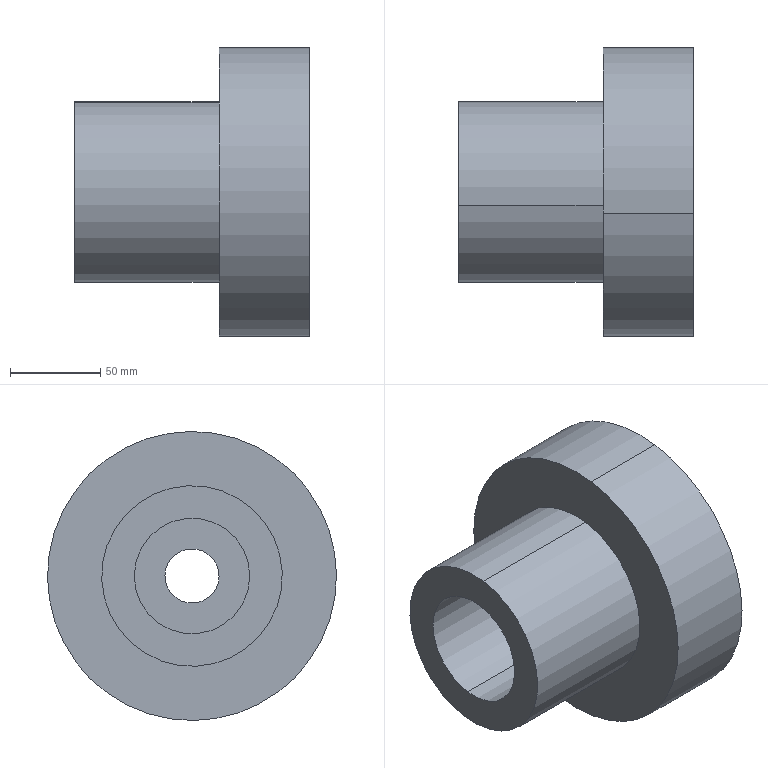Component | SolidWorks | Piston-1 | 1 solid | 18 faces | box 130 x 160 x 160 mm | volume 1255299 mm3 | cylinder 12 | plane 6 | commonest cylinder face diameters 100 x4 30 x2 34 x2 160 x2 64 x2
build123d program:
from build123d import *

# Parameters (mm, degrees)
M30_TAPPED_HOLE1_D     = 30
M30_TAPPED_HOLE1_DEPTH = 115


with BuildPart() as part:
    # Sketch1 → Revolve1 (revolve)
    with BuildSketch(Plane(origin=(0, 0, 0), x_dir=(1, 0, 0), z_dir=(0, 1, 0))):
        Polygon((10, 61), (32, 61), (32, 130), (50, 130), (50, 50), (80, 50), (80, 0), (50, 0), (50, 15), (17, 15), (17, 45), (10, 45), align=None)
    revolve(axis=Axis((0, 0, 0), (0, 0, -1)))

    # M30 Tapped Hole1
    with Locations(Plane.XY.offset(-15)):
        with Locations((0, 0)):
            Hole(M30_TAPPED_HOLE1_D / 2, depth=M30_TAPPED_HOLE1_DEPTH)


solid = part.part

# Placed as in the assembly
solid = solid.moved(Location((-28.66, 0, 0), (0, 90, 0)))
STEP:
#1=CARTESIAN_POINT('',(-3.53,0.08713,-0.5841));
#2=VERTEX_POINT('',#1);
#3=CARTESIAN_POINT('',(-3.53,-0.08713,0.5841));
#4=VERTEX_POINT('',#3);
#5=CARTESIAN_POINT('',(-3.53,-0.,0.));
#6=DIRECTION('',(-1.,-0.,0.));
#7=DIRECTION('',(0.,-0.1475,0.9891));
#8=AXIS2_PLACEMENT_3D('',#5,#6,#7);
#9=CIRCLE('',#8,0.5906);
#10=EDGE_CURVE('',#2,#4,#9,.T.);
#11=ORIENTED_EDGE('',*,*,#10,.T.);
#12=CARTESIAN_POINT('',(-2.9,-0.08713,0.5841));
#13=VERTEX_POINT('',#12);
#14=CARTESIAN_POINT('',(-1.719,-0.08713,0.5841));
#15=DIRECTION('',(1.,0.,-0.));
#16=VECTOR('',#15,39.37);
#17=LINE('',#14,#16);
#18=EDGE_CURVE('',#4,#13,#17,.T.);
#19=ORIENTED_EDGE('',*,*,#18,.T.);
#20=CARTESIAN_POINT('',(-2.9,0.08713,-0.5841));
#21=VERTEX_POINT('',#20);
#22=CARTESIAN_POINT('',(-2.9,-0.,0.));
#23=DIRECTION('',(1.,0.,-0.));
#24=DIRECTION('',(-0.,0.1475,-0.9891));
#25=AXIS2_PLACEMENT_3D('',#22,#23,#24);
#26=CIRCLE('',#25,0.5906);
#27=EDGE_CURVE('',#13,#21,#26,.T.);
#28=ORIENTED_EDGE('',*,*,#27,.T.);
#29=CARTESIAN_POINT('',(-1.719,0.08713,-0.5841));
#30=DIRECTION('',(1.,0.,-0.));
#31=VECTOR('',#30,39.37);
#32=LINE('',#29,#31);
#33=EDGE_CURVE('',#2,#21,#32,.T.);
#34=ORIENTED_EDGE('',*,*,#33,.F.);
#35=EDGE_LOOP('',(#11,#19,#28,#34));
#36=FACE_OUTER_BOUND('',#35,.T.);
#37=CARTESIAN_POINT('',(-1.719,-0.,0.));
#38=DIRECTION('',(1.,0.,-0.));
#39=DIRECTION('',(-0.,0.1475,-0.9891));
#40=AXIS2_PLACEMENT_3D('',#37,#38,#39);
#41=CYLINDRICAL_SURFACE('',#40,0.5906);
#42=ADVANCED_FACE('',(#36),#41,.F.);
#43=CARTESIAN_POINT('',(-2.9,-0.09875,0.662));
#44=VERTEX_POINT('',#43);
#45=CARTESIAN_POINT('',(-2.9,0.09875,-0.662));
#46=VERTEX_POINT('',#45);
#47=CARTESIAN_POINT('',(-2.9,-0.,0.));
#48=DIRECTION('',(1.,0.,-0.));
#49=DIRECTION('',(-0.,0.1475,-0.9891));
#50=AXIS2_PLACEMENT_3D('',#47,#48,#49);
#51=CIRCLE('',#50,0.6693);
#52=EDGE_CURVE('',#44,#46,#51,.T.);
#53=ORIENTED_EDGE('',*,*,#52,.F.);
#54=CARTESIAN_POINT('',(-1.719,-0.09875,0.662));
#55=VERTEX_POINT('',#54);
#56=CARTESIAN_POINT('',(-1.128,-0.09875,0.662));
#57=DIRECTION('',(1.,0.,-0.));
#58=VECTOR('',#57,39.37);
#59=LINE('',#56,#58);
#60=EDGE_CURVE('',#44,#55,#59,.T.);
#61=ORIENTED_EDGE('',*,*,#60,.T.);
#62=CARTESIAN_POINT('',(-1.719,0.09875,-0.662));
#63=VERTEX_POINT('',#62);
#64=CARTESIAN_POINT('',(-1.719,-0.,0.));
#65=DIRECTION('',(1.,0.,-0.));
#66=DIRECTION('',(-0.,0.1475,-0.9891));
#67=AXIS2_PLACEMENT_3D('',#64,#65,#66);
#68=CIRCLE('',#67,0.6693);
#69=EDGE_CURVE('',#55,#63,#68,.T.);
#70=ORIENTED_EDGE('',*,*,#69,.T.);
#71=CARTESIAN_POINT('',(-1.128,0.09875,-0.662));
#72=DIRECTION('',(1.,0.,-0.));
#73=VECTOR('',#72,39.37);
#74=LINE('',#71,#73);
#75=EDGE_CURVE('',#46,#63,#74,.T.);
#76=ORIENTED_EDGE('',*,*,#75,.F.);
#77=EDGE_LOOP('',(#53,#61,#70,#76));
#78=FACE_OUTER_BOUND('',#77,.T.);
#79=CARTESIAN_POINT('',(-1.128,-0.,-0.));
#80=DIRECTION('',(1.,0.,-0.));
#81=DIRECTION('',(-0.,0.1475,-0.9891));
#82=AXIS2_PLACEMENT_3D('',#79,#80,#81);
#83=CYLINDRICAL_SURFACE('',#82,0.6693);
#84=ADVANCED_FACE('',(#78),#83,.F.);
#85=CARTESIAN_POINT('',(-1.719,-0.2904,1.947));
#86=VERTEX_POINT('',#85);
#87=CARTESIAN_POINT('',(-1.719,0.2904,-1.947));
#88=VERTEX_POINT('',#87);
#89=CARTESIAN_POINT('',(-1.719,-0.,0.));
#90=DIRECTION('',(1.,0.,-0.));
#91=DIRECTION('',(-0.,0.1475,-0.9891));
#92=AXIS2_PLACEMENT_3D('',#89,#90,#91);
#93=CIRCLE('',#92,1.969);
#94=EDGE_CURVE('',#86,#88,#93,.T.);
#95=ORIENTED_EDGE('',*,*,#94,.F.);
#96=CARTESIAN_POINT('',(-1.128,-0.2904,1.947));
#97=VERTEX_POINT('',#96);
#98=CARTESIAN_POINT('',(-1.128,-0.2904,1.947));
#99=DIRECTION('',(1.,0.,-0.));
#100=VECTOR('',#99,39.37);
#101=LINE('',#98,#100);
#102=EDGE_CURVE('',#86,#97,#101,.T.);
#103=ORIENTED_EDGE('',*,*,#102,.T.);
#104=CARTESIAN_POINT('',(-1.128,0.2904,-1.947));
#105=VERTEX_POINT('',#104);
#106=CARTESIAN_POINT('',(-1.128,-0.,-0.));
#107=DIRECTION('',(1.,0.,-0.));
#108=DIRECTION('',(-0.,0.1475,-0.9891));
#109=AXIS2_PLACEMENT_3D('',#106,#107,#108);
#110=CIRCLE('',#109,1.969);
#111=EDGE_CURVE('',#97,#105,#110,.T.);
#112=ORIENTED_EDGE('',*,*,#111,.T.);
#113=CARTESIAN_POINT('',(-1.128,0.2904,-1.947));
#114=DIRECTION('',(1.,0.,-0.));
#115=VECTOR('',#114,39.37);
#116=LINE('',#113,#115);
#117=EDGE_CURVE('',#88,#105,#116,.T.);
#118=ORIENTED_EDGE('',*,*,#117,.F.);
#119=EDGE_LOOP('',(#95,#103,#112,#118));
#120=FACE_OUTER_BOUND('',#119,.T.);
#121=CARTESIAN_POINT('',(-1.128,-0.,-0.));
#122=DIRECTION('',(1.,0.,-0.));
#123=DIRECTION('',(-0.,0.1475,-0.9891));
#124=AXIS2_PLACEMENT_3D('',#121,#122,#123);
#125=CYLINDRICAL_SURFACE('',#124,1.969);
#126=ADVANCED_FACE('',(#120),#125,.F.);
#127=CARTESIAN_POINT('',(-3.097,0.4647,-3.115));
#128=VERTEX_POINT('',#127);
#129=CARTESIAN_POINT('',(-3.097,-0.4647,3.115));
#130=VERTEX_POINT('',#129);
#131=CARTESIAN_POINT('',(-3.097,-0.,0.));
#132=DIRECTION('',(1.,0.,-0.));
#133=DIRECTION('',(-0.,0.1475,-0.9891));
#134=AXIS2_PLACEMENT_3D('',#131,#132,#133);
#135=CIRCLE('',#134,3.15);
#136=EDGE_CURVE('',#128,#130,#135,.T.);
#137=ORIENTED_EDGE('',*,*,#136,.T.);
#138=CARTESIAN_POINT('',(-1.128,-0.4647,3.115));
#139=VERTEX_POINT('',#138);
#140=CARTESIAN_POINT('',(-1.128,-0.4647,3.115));
#141=DIRECTION('',(1.,0.,-0.));
#142=VECTOR('',#141,39.37);
#143=LINE('',#140,#142);
#144=EDGE_CURVE('',#130,#139,#143,.T.);
#145=ORIENTED_EDGE('',*,*,#144,.T.);
#146=CARTESIAN_POINT('',(-1.128,0.4647,-3.115));
#147=VERTEX_POINT('',#146);
#148=CARTESIAN_POINT('',(-1.128,-0.,-0.));
#149=DIRECTION('',(1.,0.,-0.));
#150=DIRECTION('',(-0.,0.1475,-0.9891));
#151=AXIS2_PLACEMENT_3D('',#148,#149,#150);
#152=CIRCLE('',#151,3.15);
#153=EDGE_CURVE('',#147,#139,#152,.T.);
#154=ORIENTED_EDGE('',*,*,#153,.F.);
#155=CARTESIAN_POINT('',(-1.128,0.4647,-3.115));
#156=DIRECTION('',(1.,0.,-0.));
#157=VECTOR('',#156,39.37);
#158=LINE('',#155,#157);
#159=EDGE_CURVE('',#128,#147,#158,.T.);
#160=ORIENTED_EDGE('',*,*,#159,.F.);
#161=EDGE_LOOP('',(#137,#145,#154,#160));
#162=FACE_OUTER_BOUND('',#161,.T.);
#163=CARTESIAN_POINT('',(-1.128,-0.,-0.));
#164=DIRECTION('',(1.,0.,-0.));
#165=DIRECTION('',(-0.,0.1475,-0.9891));
#166=AXIS2_PLACEMENT_3D('',#163,#164,#165);
#167=CYLINDRICAL_SURFACE('',#166,3.15);
#168=ADVANCED_FACE('',(#162),#167,.T.);
#169=CARTESIAN_POINT('',(-6.246,0.2904,-1.947));
#170=VERTEX_POINT('',#169);
#171=CARTESIAN_POINT('',(-6.246,-0.2904,1.947));
#172=VERTEX_POINT('',#171);
#173=CARTESIAN_POINT('',(-6.246,-0.,0.));
#174=DIRECTION('',(1.,0.,-0.));
#175=DIRECTION('',(-0.,0.1475,-0.9891));
#176=AXIS2_PLACEMENT_3D('',#173,#174,#175);
#177=CIRCLE('',#176,1.969);
#178=EDGE_CURVE('',#170,#172,#177,.T.);
#179=ORIENTED_EDGE('',*,*,#178,.T.);
#180=CARTESIAN_POINT('',(-3.097,-0.2904,1.947));
#181=VERTEX_POINT('',#180);
#182=CARTESIAN_POINT('',(-1.128,-0.2904,1.947));
#183=DIRECTION('',(1.,0.,-0.));
#184=VECTOR('',#183,39.37);
#185=LINE('',#182,#184);
#186=EDGE_CURVE('',#172,#181,#185,.T.);
#187=ORIENTED_EDGE('',*,*,#186,.T.);
#188=CARTESIAN_POINT('',(-3.097,0.2904,-1.947));
#189=VERTEX_POINT('',#188);
#190=CARTESIAN_POINT('',(-3.097,-0.,0.));
#191=DIRECTION('',(1.,0.,-0.));
#192=DIRECTION('',(-0.,0.1475,-0.9891));
#193=AXIS2_PLACEMENT_3D('',#190,#191,#192);
#194=CIRCLE('',#193,1.969);
#195=EDGE_CURVE('',#189,#181,#194,.T.);
#196=ORIENTED_EDGE('',*,*,#195,.F.);
#197=CARTESIAN_POINT('',(-1.128,0.2904,-1.947));
#198=DIRECTION('',(1.,0.,-0.));
#199=VECTOR('',#198,39.37);
#200=LINE('',#197,#199);
#201=EDGE_CURVE('',#170,#189,#200,.T.);
#202=ORIENTED_EDGE('',*,*,#201,.F.);
#203=EDGE_LOOP('',(#179,#187,#196,#202));
#204=FACE_OUTER_BOUND('',#203,.T.);
#205=CARTESIAN_POINT('',(-1.128,-0.,-0.));
#206=DIRECTION('',(1.,0.,-0.));
#207=DIRECTION('',(-0.,0.1475,-0.9891));
#208=AXIS2_PLACEMENT_3D('',#205,#206,#207);
#209=CYLINDRICAL_SURFACE('',#208,1.969);
#210=ADVANCED_FACE('',(#204),#209,.T.);
#211=CARTESIAN_POINT('',(-6.246,-0.1859,1.246));
#212=VERTEX_POINT('',#211);
#213=CARTESIAN_POINT('',(-6.246,0.1859,-1.246));
#214=VERTEX_POINT('',#213);
#215=CARTESIAN_POINT('',(-6.246,-0.,0.));
#216=DIRECTION('',(1.,0.,-0.));
#217=DIRECTION('',(-0.,0.1475,-0.9891));
#218=AXIS2_PLACEMENT_3D('',#215,#216,#217);
#219=CIRCLE('',#218,1.26);
#220=EDGE_CURVE('',#212,#214,#219,.T.);
#221=ORIENTED_EDGE('',*,*,#220,.F.);
#222=CARTESIAN_POINT('',(-3.53,-0.1859,1.246));
#223=VERTEX_POINT('',#222);
#224=CARTESIAN_POINT('',(-1.128,-0.1859,1.246));
#225=DIRECTION('',(1.,0.,-0.));
#226=VECTOR('',#225,39.37);
#227=LINE('',#224,#226);
#228=EDGE_CURVE('',#212,#223,#227,.T.);
#229=ORIENTED_EDGE('',*,*,#228,.T.);
#230=CARTESIAN_POINT('',(-3.53,0.1859,-1.246));
#231=VERTEX_POINT('',#230);
#232=CARTESIAN_POINT('',(-3.53,-0.,0.));
#233=DIRECTION('',(1.,0.,-0.));
#234=DIRECTION('',(-0.,0.1475,-0.9891));
#235=AXIS2_PLACEMENT_3D('',#232,#233,#234);
#236=CIRCLE('',#235,1.26);
#237=EDGE_CURVE('',#223,#231,#236,.T.);
#238=ORIENTED_EDGE('',*,*,#237,.T.);
#239=CARTESIAN_POINT('',(-1.128,0.1859,-1.246));
#240=DIRECTION('',(1.,0.,-0.));
#241=VECTOR('',#240,39.37);
#242=LINE('',#239,#241);
#243=EDGE_CURVE('',#214,#231,#242,.T.);
#244=ORIENTED_EDGE('',*,*,#243,.F.);
#245=EDGE_LOOP('',(#221,#229,#238,#244));
#246=FACE_OUTER_BOUND('',#245,.T.);
#247=CARTESIAN_POINT('',(-1.128,-0.,-0.));
#248=DIRECTION('',(1.,0.,-0.));
#249=DIRECTION('',(-0.,0.1475,-0.9891));
#250=AXIS2_PLACEMENT_3D('',#247,#248,#249);
#251=CYLINDRICAL_SURFACE('',#250,1.26);
#252=ADVANCED_FACE('',(#246),#251,.F.);
#253=ORIENTED_EDGE('',*,*,#10,.F.);
#254=CARTESIAN_POINT('',(-3.53,-0.,0.));
#255=DIRECTION('',(-1.,-0.,0.));
#256=DIRECTION('',(0.,-0.1475,0.9891));
#257=AXIS2_PLACEMENT_3D('',#254,#255,#256);
#258=CIRCLE('',#257,0.5906);
#259=EDGE_CURVE('',#4,#2,#258,.T.);
#260=ORIENTED_EDGE('',*,*,#259,.F.);
#261=EDGE_LOOP('',(#253,#260));
#262=FACE_BOUND('',#261,.T.);
#263=CARTESIAN_POINT('',(-3.53,-0.,0.));
#264=DIRECTION('',(1.,0.,-0.));
#265=DIRECTION('',(-0.,0.1475,-0.9891));
#266=AXIS2_PLACEMENT_3D('',#263,#264,#265);
#267=CIRCLE('',#266,1.26);
#268=EDGE_CURVE('',#231,#223,#267,.T.);
#269=ORIENTED_EDGE('',*,*,#268,.F.);
#270=ORIENTED_EDGE('',*,*,#237,.F.);
#271=EDGE_LOOP('',(#269,#270));
#272=FACE_OUTER_BOUND('',#271,.T.);
#273=CARTESIAN_POINT('',(-3.53,0.05809,-0.3894));
#274=DIRECTION('',(-1.,-0.,0.));
#275=DIRECTION('',(0.,-0.1475,0.9891));
#276=AXIS2_PLACEMENT_3D('',#273,#274,#275);
#277=PLANE('',#276);
#278=ADVANCED_FACE('',(#262,#272),#277,.T.);
#279=ORIENTED_EDGE('',*,*,#228,.F.);
#280=CARTESIAN_POINT('',(-6.246,-0.,0.));
#281=DIRECTION('',(1.,0.,-0.));
#282=DIRECTION('',(-0.,0.1475,-0.9891));
#283=AXIS2_PLACEMENT_3D('',#280,#281,#282);
#284=CIRCLE('',#283,1.26);
#285=EDGE_CURVE('',#214,#212,#284,.T.);
#286=ORIENTED_EDGE('',*,*,#285,.F.);
#287=ORIENTED_EDGE('',*,*,#243,.T.);
#288=ORIENTED_EDGE('',*,*,#268,.T.);
#289=EDGE_LOOP('',(#279,#286,#287,#288));
#290=FACE_OUTER_BOUND('',#289,.T.);
#291=CARTESIAN_POINT('',(-1.128,-0.,-0.));
#292=DIRECTION('',(1.,0.,-0.));
#293=DIRECTION('',(-0.,0.1475,-0.9891));
#294=AXIS2_PLACEMENT_3D('',#291,#292,#293);
#295=CYLINDRICAL_SURFACE('',#294,1.26);
#296=ADVANCED_FACE('',(#290),#295,.F.);
#297=ORIENTED_EDGE('',*,*,#285,.T.);
#298=ORIENTED_EDGE('',*,*,#220,.T.);
#299=EDGE_LOOP('',(#297,#298));
#300=FACE_BOUND('',#299,.T.);
#301=ORIENTED_EDGE('',*,*,#178,.F.);
#302=CARTESIAN_POINT('',(-6.246,-0.,0.));
#303=DIRECTION('',(1.,0.,-0.));
#304=DIRECTION('',(-0.,0.1475,-0.9891));
#305=AXIS2_PLACEMENT_3D('',#302,#303,#304);
#306=CIRCLE('',#305,1.969);
#307=EDGE_CURVE('',#172,#170,#306,.T.);
#308=ORIENTED_EDGE('',*,*,#307,.F.);
#309=EDGE_LOOP('',(#301,#308));
#310=FACE_OUTER_BOUND('',#309,.T.);
#311=CARTESIAN_POINT('',(-6.246,0.1859,-1.246));
#312=DIRECTION('',(-1.,-0.,0.));
#313=DIRECTION('',(0.,-0.1475,0.9891));
#314=AXIS2_PLACEMENT_3D('',#311,#312,#313);
#315=PLANE('',#314);
#316=ADVANCED_FACE('',(#300,#310),#315,.T.);
#317=ORIENTED_EDGE('',*,*,#186,.F.);
#318=ORIENTED_EDGE('',*,*,#307,.T.);
#319=ORIENTED_EDGE('',*,*,#201,.T.);
#320=CARTESIAN_POINT('',(-3.097,-0.,0.));
#321=DIRECTION('',(1.,0.,-0.));
#322=DIRECTION('',(-0.,0.1475,-0.9891));
#323=AXIS2_PLACEMENT_3D('',#320,#321,#322);
#324=CIRCLE('',#323,1.969);
#325=EDGE_CURVE('',#181,#189,#324,.T.);
#326=ORIENTED_EDGE('',*,*,#325,.F.);
#327=EDGE_LOOP('',(#317,#318,#319,#326));
#328=FACE_OUTER_BOUND('',#327,.T.);
#329=CARTESIAN_POINT('',(-1.128,-0.,-0.));
#330=DIRECTION('',(1.,0.,-0.));
#331=DIRECTION('',(-0.,0.1475,-0.9891));
#332=AXIS2_PLACEMENT_3D('',#329,#330,#331);
#333=CYLINDRICAL_SURFACE('',#332,1.969);
#334=ADVANCED_FACE('',(#328),#333,.T.);
#335=ORIENTED_EDGE('',*,*,#195,.T.);
#336=ORIENTED_EDGE('',*,*,#325,.T.);
#337=EDGE_LOOP('',(#335,#336));
#338=FACE_BOUND('',#337,.T.);
#339=ORIENTED_EDGE('',*,*,#136,.F.);
#340=CARTESIAN_POINT('',(-3.097,-0.,0.));
#341=DIRECTION('',(1.,0.,-0.));
#342=DIRECTION('',(-0.,0.1475,-0.9891));
#343=AXIS2_PLACEMENT_3D('',#340,#341,#342);
#344=CIRCLE('',#343,3.15);
#345=EDGE_CURVE('',#130,#128,#344,.T.);
#346=ORIENTED_EDGE('',*,*,#345,.F.);
#347=EDGE_LOOP('',(#339,#346));
#348=FACE_OUTER_BOUND('',#347,.T.);
#349=CARTESIAN_POINT('',(-3.097,0.2904,-1.947));
#350=DIRECTION('',(-1.,-0.,0.));
#351=DIRECTION('',(0.,-0.1475,0.9891));
#352=AXIS2_PLACEMENT_3D('',#349,#350,#351);
#353=PLANE('',#352);
#354=ADVANCED_FACE('',(#338,#348),#353,.T.);
#355=ORIENTED_EDGE('',*,*,#144,.F.);
#356=ORIENTED_EDGE('',*,*,#345,.T.);
#357=ORIENTED_EDGE('',*,*,#159,.T.);
#358=CARTESIAN_POINT('',(-1.128,-0.,-0.));
#359=DIRECTION('',(1.,0.,-0.));
#360=DIRECTION('',(-0.,0.1475,-0.9891));
#361=AXIS2_PLACEMENT_3D('',#358,#359,#360);
#362=CIRCLE('',#361,3.15);
#363=EDGE_CURVE('',#139,#147,#362,.T.);
#364=ORIENTED_EDGE('',*,*,#363,.F.);
#365=EDGE_LOOP('',(#355,#356,#357,#364));
#366=FACE_OUTER_BOUND('',#365,.T.);
#367=CARTESIAN_POINT('',(-1.128,-0.,-0.));
#368=DIRECTION('',(1.,0.,-0.));
#369=DIRECTION('',(-0.,0.1475,-0.9891));
#370=AXIS2_PLACEMENT_3D('',#367,#368,#369);
#371=CYLINDRICAL_SURFACE('',#370,3.15);
#372=ADVANCED_FACE('',(#366),#371,.T.);
#373=ORIENTED_EDGE('',*,*,#153,.T.);
#374=ORIENTED_EDGE('',*,*,#363,.T.);
#375=EDGE_LOOP('',(#373,#374));
#376=FACE_OUTER_BOUND('',#375,.T.);
#377=CARTESIAN_POINT('',(-1.128,-0.,-0.));
#378=DIRECTION('',(1.,0.,-0.));
#379=DIRECTION('',(-0.,0.1475,-0.9891));
#380=AXIS2_PLACEMENT_3D('',#377,#378,#379);
#381=CIRCLE('',#380,1.969);
#382=EDGE_CURVE('',#105,#97,#381,.T.);
#383=ORIENTED_EDGE('',*,*,#382,.F.);
#384=ORIENTED_EDGE('',*,*,#111,.F.);
#385=EDGE_LOOP('',(#383,#384));
#386=FACE_BOUND('',#385,.T.);
#387=CARTESIAN_POINT('',(-1.128,0.4647,-3.115));
#388=DIRECTION('',(1.,0.,-0.));
#389=DIRECTION('',(-0.,0.1475,-0.9891));
#390=AXIS2_PLACEMENT_3D('',#387,#388,#389);
#391=PLANE('',#390);
#392=ADVANCED_FACE('',(#376,#386),#391,.T.);
#393=ORIENTED_EDGE('',*,*,#102,.F.);
#394=CARTESIAN_POINT('',(-1.719,-0.,0.));
#395=DIRECTION('',(1.,0.,-0.));
#396=DIRECTION('',(-0.,0.1475,-0.9891));
#397=AXIS2_PLACEMENT_3D('',#394,#395,#396);
#398=CIRCLE('',#397,1.969);
#399=EDGE_CURVE('',#88,#86,#398,.T.);
#400=ORIENTED_EDGE('',*,*,#399,.F.);
#401=ORIENTED_EDGE('',*,*,#117,.T.);
#402=ORIENTED_EDGE('',*,*,#382,.T.);
#403=EDGE_LOOP('',(#393,#400,#401,#402));
#404=FACE_OUTER_BOUND('',#403,.T.);
#405=CARTESIAN_POINT('',(-1.128,-0.,-0.));
#406=DIRECTION('',(1.,0.,-0.));
#407=DIRECTION('',(-0.,0.1475,-0.9891));
#408=AXIS2_PLACEMENT_3D('',#405,#406,#407);
#409=CYLINDRICAL_SURFACE('',#408,1.969);
#410=ADVANCED_FACE('',(#404),#409,.F.);
#411=ORIENTED_EDGE('',*,*,#399,.T.);
#412=ORIENTED_EDGE('',*,*,#94,.T.);
#413=EDGE_LOOP('',(#411,#412));
#414=FACE_OUTER_BOUND('',#413,.T.);
#415=CARTESIAN_POINT('',(-1.719,-0.,0.));
#416=DIRECTION('',(1.,0.,-0.));
#417=DIRECTION('',(-0.,0.1475,-0.9891));
#418=AXIS2_PLACEMENT_3D('',#415,#416,#417);
#419=CIRCLE('',#418,0.6693);
#420=EDGE_CURVE('',#63,#55,#419,.T.);
#421=ORIENTED_EDGE('',*,*,#420,.F.);
#422=ORIENTED_EDGE('',*,*,#69,.F.);
#423=EDGE_LOOP('',(#421,#422));
#424=FACE_BOUND('',#423,.T.);
#425=CARTESIAN_POINT('',(-1.719,0.2904,-1.947));
#426=DIRECTION('',(1.,0.,-0.));
#427=DIRECTION('',(-0.,0.1475,-0.9891));
#428=AXIS2_PLACEMENT_3D('',#425,#426,#427);
#429=PLANE('',#428);
#430=ADVANCED_FACE('',(#414,#424),#429,.T.);
#431=ORIENTED_EDGE('',*,*,#60,.F.);
#432=CARTESIAN_POINT('',(-2.9,-0.,0.));
#433=DIRECTION('',(1.,0.,-0.));
#434=DIRECTION('',(-0.,0.1475,-0.9891));
#435=AXIS2_PLACEMENT_3D('',#432,#433,#434);
#436=CIRCLE('',#435,0.6693);
#437=EDGE_CURVE('',#46,#44,#436,.T.);
#438=ORIENTED_EDGE('',*,*,#437,.F.);
#439=ORIENTED_EDGE('',*,*,#75,.T.);
#440=ORIENTED_EDGE('',*,*,#420,.T.);
#441=EDGE_LOOP('',(#431,#438,#439,#440));
#442=FACE_OUTER_BOUND('',#441,.T.);
#443=CARTESIAN_POINT('',(-1.128,-0.,-0.));
#444=DIRECTION('',(1.,0.,-0.));
#445=DIRECTION('',(-0.,0.1475,-0.9891));
#446=AXIS2_PLACEMENT_3D('',#443,#444,#445);
#447=CYLINDRICAL_SURFACE('',#446,0.6693);
#448=ADVANCED_FACE('',(#442),#447,.F.);
#449=CARTESIAN_POINT('',(-2.9,-0.,0.));
#450=DIRECTION('',(1.,0.,-0.));
#451=DIRECTION('',(-0.,0.1475,-0.9891));
#452=AXIS2_PLACEMENT_3D('',#449,#450,#451);
#453=CIRCLE('',#452,0.5906);
#454=EDGE_CURVE('',#21,#13,#453,.T.);
#455=ORIENTED_EDGE('',*,*,#454,.F.);
#456=ORIENTED_EDGE('',*,*,#27,.F.);
#457=EDGE_LOOP('',(#455,#456));
#458=FACE_BOUND('',#457,.T.);
#459=ORIENTED_EDGE('',*,*,#437,.T.);
#460=ORIENTED_EDGE('',*,*,#52,.T.);
#461=EDGE_LOOP('',(#459,#460));
#462=FACE_OUTER_BOUND('',#461,.T.);
#463=CARTESIAN_POINT('',(-2.9,0.05809,-0.3894));
#464=DIRECTION('',(1.,0.,-0.));
#465=DIRECTION('',(-0.,0.1475,-0.9891));
#466=AXIS2_PLACEMENT_3D('',#463,#464,#465);
#467=PLANE('',#466);
#468=ADVANCED_FACE('',(#458,#462),#467,.T.);
#469=ORIENTED_EDGE('',*,*,#18,.F.);
#470=ORIENTED_EDGE('',*,*,#259,.T.);
#471=ORIENTED_EDGE('',*,*,#33,.T.);
#472=ORIENTED_EDGE('',*,*,#454,.T.);
#473=EDGE_LOOP('',(#469,#470,#471,#472));
#474=FACE_OUTER_BOUND('',#473,.T.);
#475=CARTESIAN_POINT('',(-1.719,-0.,0.));
#476=DIRECTION('',(1.,0.,-0.));
#477=DIRECTION('',(-0.,0.1475,-0.9891));
#478=AXIS2_PLACEMENT_3D('',#475,#476,#477);
#479=CYLINDRICAL_SURFACE('',#478,0.5906);
#480=ADVANCED_FACE('',(#474),#479,.F.);
#481=CLOSED_SHELL('',(#42,#84,#126,#168,#210,#252,#278,#296,#316,#334,#354,#372,#392,#410,#430,#448,#468,#480));
#482=MANIFOLD_SOLID_BREP('',#481);
#483=CARTESIAN_POINT('',(0.,0.,0.));
#484=DIRECTION('',(0.,0.,1.));
#485=DIRECTION('',(1.,0.,0.));
#486=AXIS2_PLACEMENT_3D('',#483,#484,#485);
#487=(LENGTH_UNIT()NAMED_UNIT(*)SI_UNIT($,.METRE.));
#488=LENGTH_MEASURE_WITH_UNIT(LENGTH_MEASURE(0.0254),#487);
#489=DIMENSIONAL_EXPONENTS(1.,0.,0.,0.,0.,0.,0.);
#490=(CONVERSION_BASED_UNIT('',#488)LENGTH_UNIT()NAMED_UNIT(#489));
#491=UNCERTAINTY_MEASURE_WITH_UNIT(LENGTH_MEASURE(0.00001),#490,'','');
#492=(NAMED_UNIT(*)PLANE_ANGLE_UNIT()SI_UNIT($,.RADIAN.));
#493=(NAMED_UNIT(*)SI_UNIT($,.STERADIAN.)SOLID_ANGLE_UNIT());
#494=(GEOMETRIC_REPRESENTATION_CONTEXT(3)GLOBAL_UNCERTAINTY_ASSIGNED_CONTEXT((#491))GLOBAL_UNIT_ASSIGNED_CONTEXT((#490,#492,#493))REPRESENTATION_CONTEXT('',''));
#495=ADVANCED_BREP_SHAPE_REPRESENTATION('',(#482,#486),#494);
#496=COLOUR_RGB('',0.7922,0.8196,0.9333);
#497=FILL_AREA_STYLE_COLOUR('',#496);
#498=FILL_AREA_STYLE('',(#497));
#499=SURFACE_STYLE_FILL_AREA(#498);
#500=SURFACE_SIDE_STYLE('',(#499));
#501=SURFACE_STYLE_USAGE(.BOTH.,#500);
#502=PRESENTATION_STYLE_ASSIGNMENT((#501));
#503=STYLED_ITEM('',(#502),#482);
#504=PRESENTATION_LAYER_ASSIGNMENT('','',(#503));
#505=(LENGTH_UNIT()NAMED_UNIT(*)SI_UNIT($,.METRE.));
#506=LENGTH_MEASURE_WITH_UNIT(LENGTH_MEASURE(0.0254),#505);
#507=DIMENSIONAL_EXPONENTS(1.,0.,0.,0.,0.,0.,0.);
#508=(CONVERSION_BASED_UNIT('',#506)LENGTH_UNIT()NAMED_UNIT(#507));
#509=UNCERTAINTY_MEASURE_WITH_UNIT(LENGTH_MEASURE(0.00001),#508,'','');
#510=(NAMED_UNIT(*)PLANE_ANGLE_UNIT()SI_UNIT($,.RADIAN.));
#511=(NAMED_UNIT(*)SI_UNIT($,.STERADIAN.)SOLID_ANGLE_UNIT());
#512=(GEOMETRIC_REPRESENTATION_CONTEXT(3)GLOBAL_UNCERTAINTY_ASSIGNED_CONTEXT((#509))GLOBAL_UNIT_ASSIGNED_CONTEXT((#508,#510,#511))REPRESENTATION_CONTEXT('',''));
#513=MECHANICAL_DESIGN_GEOMETRIC_PRESENTATION_REPRESENTATION('',(#503),#512);